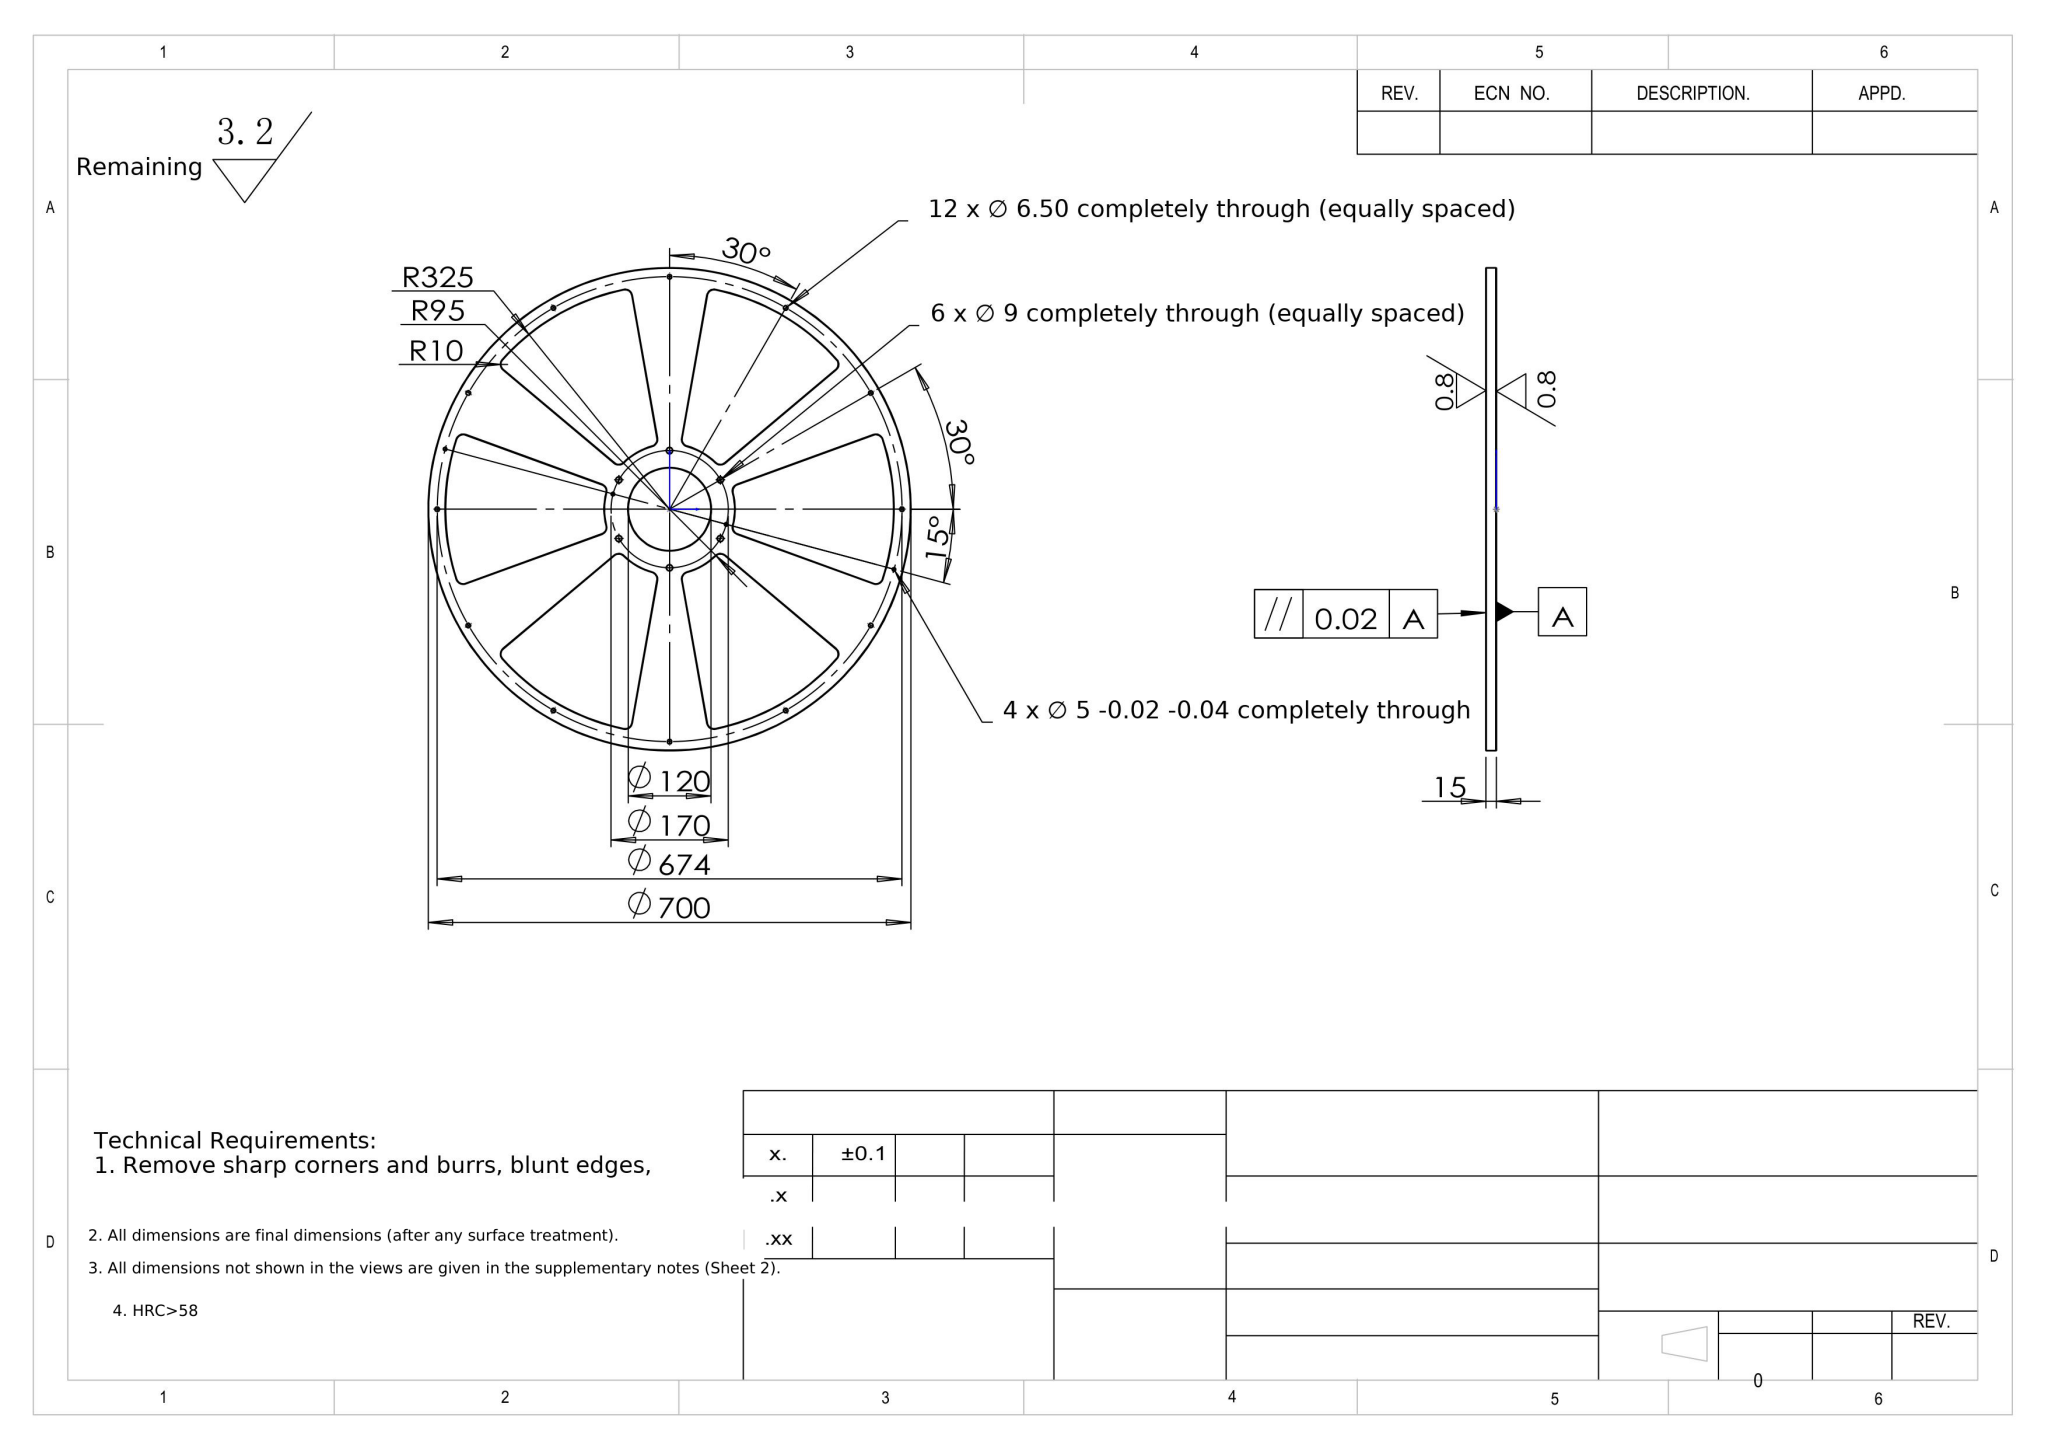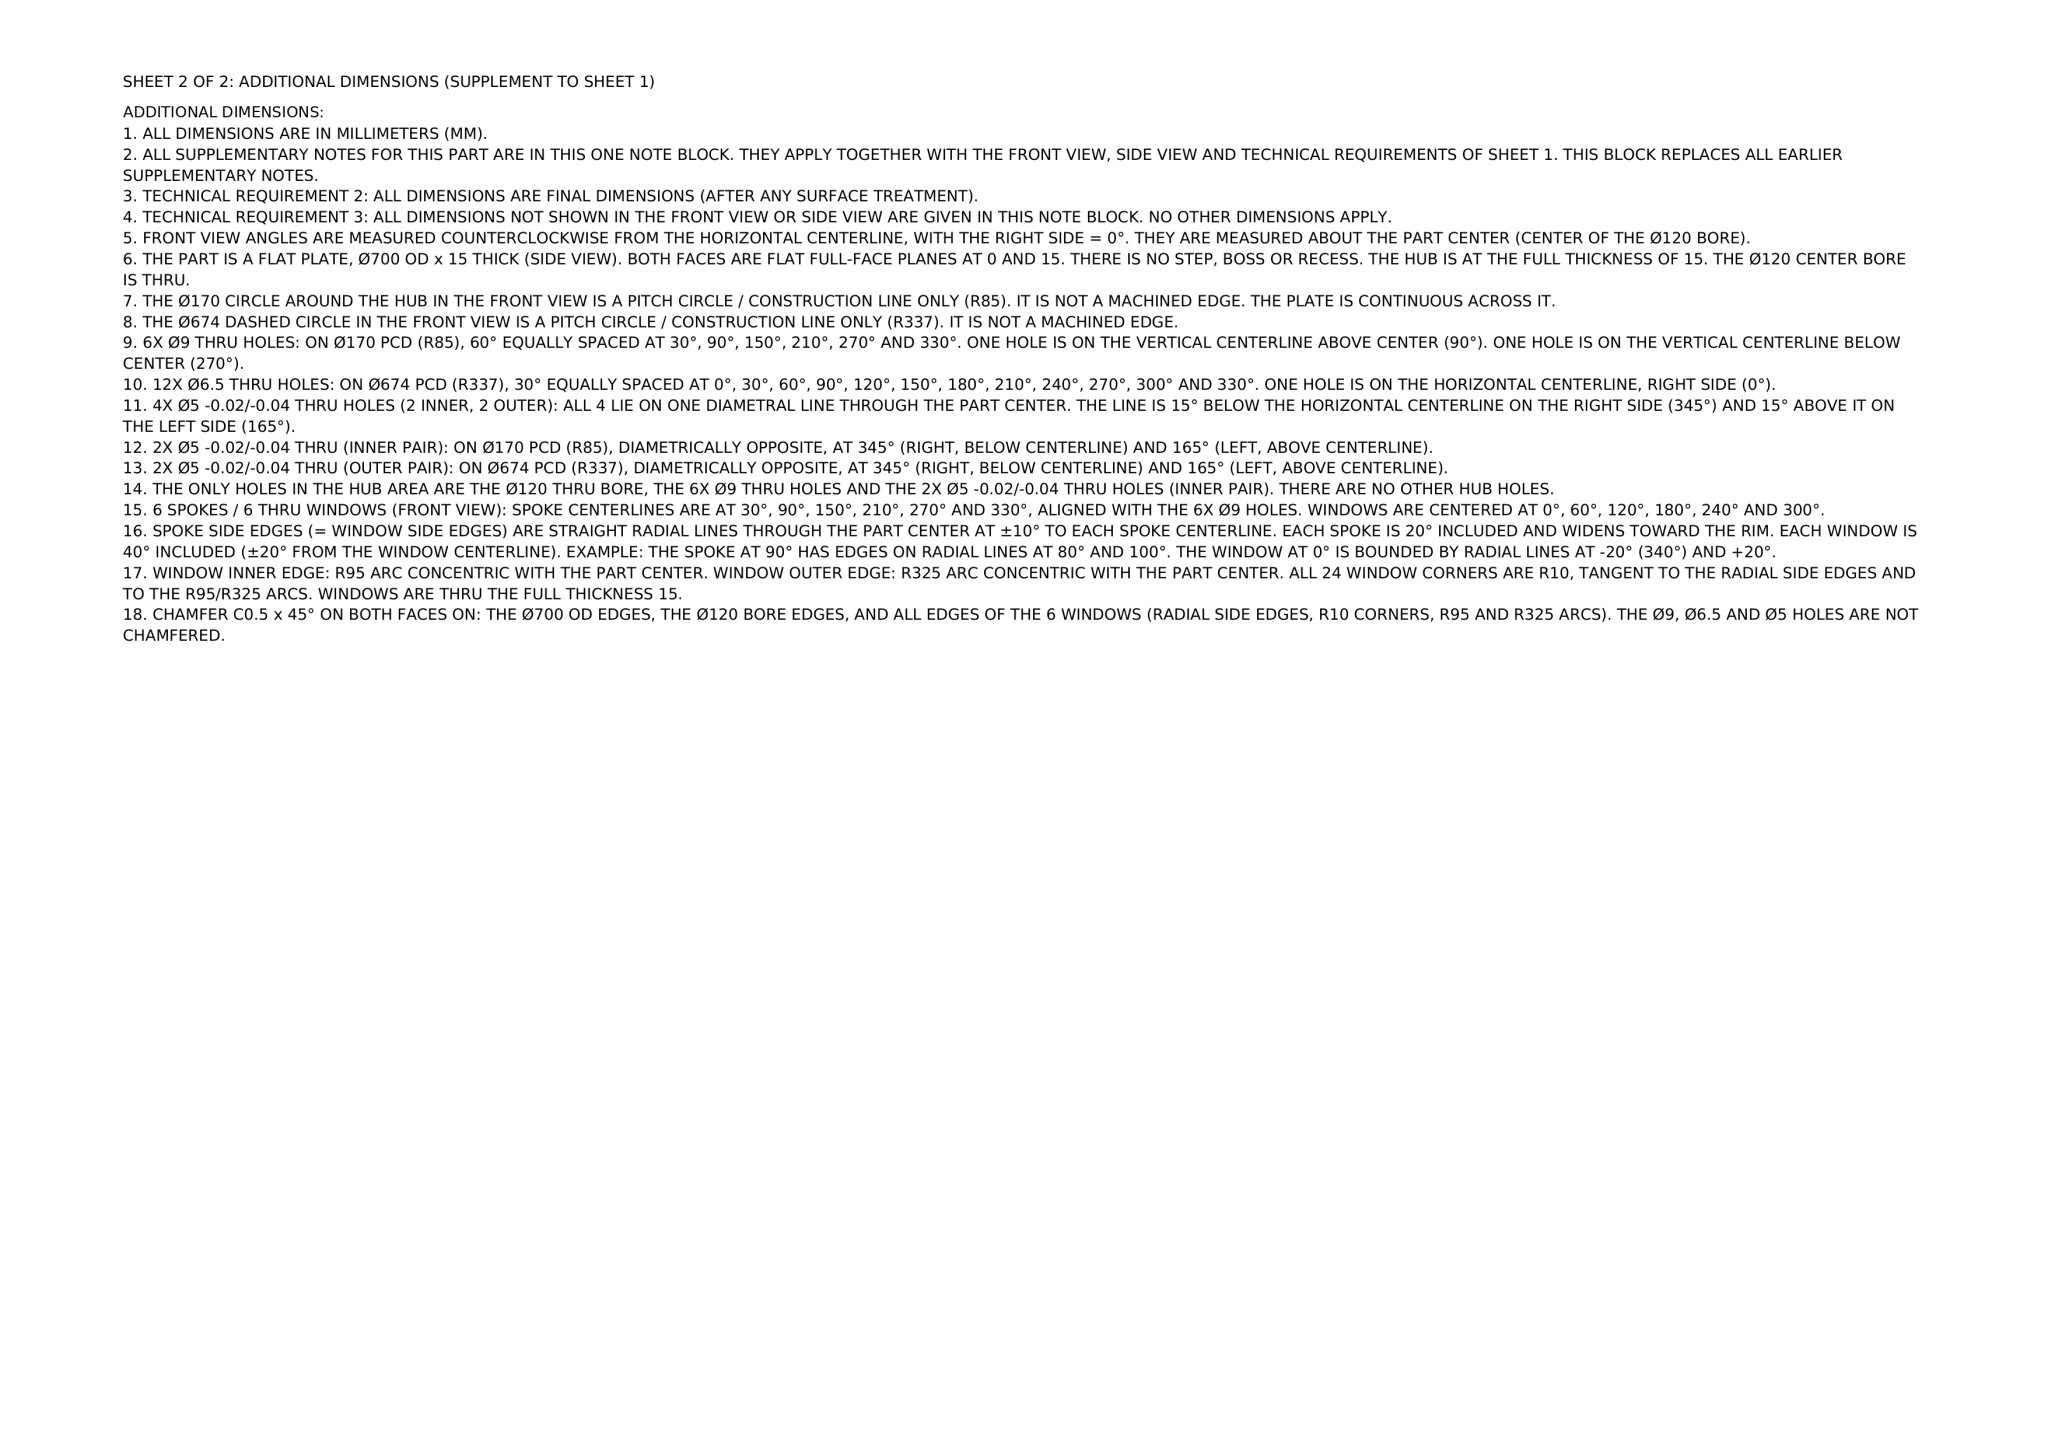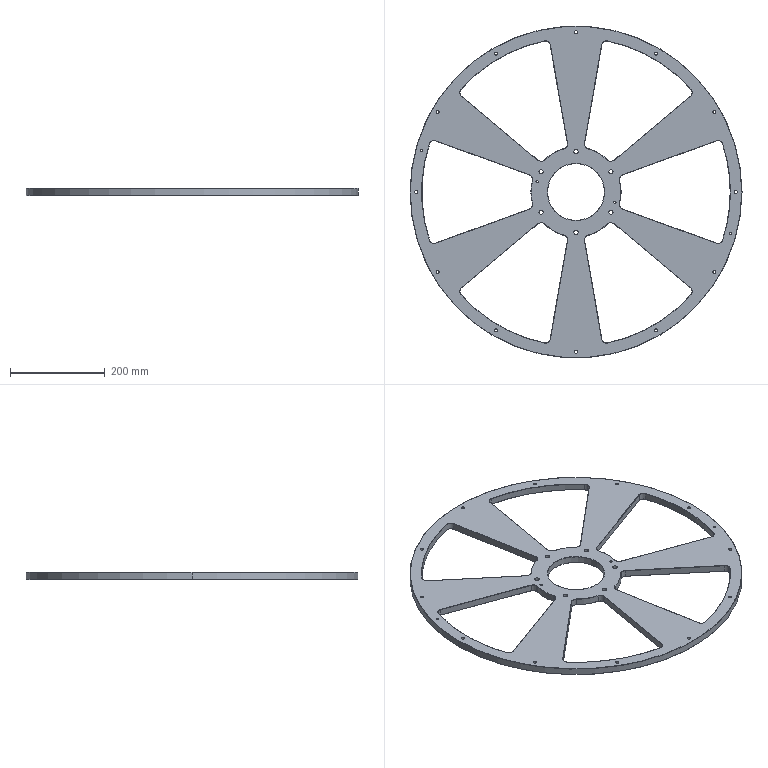Part | NX | mm | 1 solid | 226 faces | box 700 x 700 x 15 mm | volume 2560998 mm3 | cone 96 | cylinder 92 | plane 38 | commonest cylinder face diameters 20 x30 6.5 x24 9 x12 5 x8 190 x7 650 x7 120 x2 700 x2